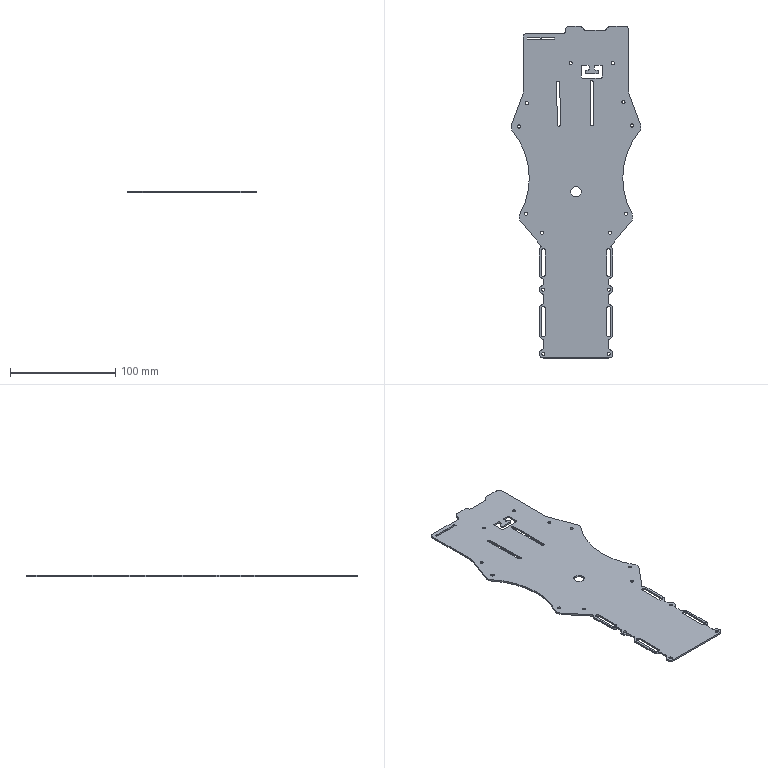Component | SolidWorks | LowerPlate-1 | 1 solid | 168 faces | box 123.18 x 315.5 x 1.6 mm | volume 42538 mm3 | cylinder 111 | plane 57 | commonest cylinder face diameters 3 x33 4 x24 2 x19 8 x18 13 x6 5 x4 140 x3 10 x2
build123d program:
from build123d import *

# Parameters (mm, degrees)
BOSS_EXTRUDE1_DEPTH  = 1.6
FILLET1_R            = 10
FILLET2_R            = 2
BOSS_EXTRUDE2_DEPTH  = 1.6
SKETCH4_R            = 5
SKETCH4_R_2          = 1.5
CUT_EXTRUDE1_2_DEPTH = 1.6
SKETCH5_R            = 1.5
CUT_EXTRUDE2_DEPTH   = 1.6
FILLET3_R            = 1
SKETCH1_W            = 1.25
SKETCH1_H            = 1.5
SKETCH1_W_2          = 1.4
CUT_EXTRUDE1_DEPTH   = 5


with BuildPart() as part:
    # Sketch1_2 → Boss-Extrude1 (new body)
    with BuildSketch(Plane.XY):
        with BuildLine():
            Line((-31, 0), (31, 0))
            ThreePointArc((31, 0), (35, 4), (31, 8))
            Line((31, 8), (31, 18))
            ThreePointArc((31, 18), (33.828, 19.172), (35, 22))
            Line((35, 22), (35, 47))
            ThreePointArc((35, 47), (33.828, 49.828), (31, 51))
            Line((31, 51), (31, 61))
            ThreePointArc((31, 61), (35, 65), (31, 69))
            Line((31, 69), (31, 75.5))
            ThreePointArc((31, 75.5), (33.828, 76.672), (35, 79.5))
            Line((35, 79.5), (35, 101.75))
            ThreePointArc((35, 101.75), (34.694, 103.284), (33.824, 104.583))
            ThreePointArc((33.824, 104.583), (33.237, 105.911), (33.703, 107.286))
            Line((33.703, 107.286), (52.509, 129.698))
            ThreePointArc((52.509, 129.698), (54, 133.254), (53.213, 137.03))
            ThreePointArc((53.213, 137.03), (44.691, 177.172), (60.131, 215.192))
            ThreePointArc((60.131, 215.192), (61.5, 218.215), (61.199, 221.519))
            Line((61.199, 221.519), (50, 252.287))
            Line((50, 252.287), (50, 308))
            Line((50, 308), (-50, 308))
            Line((-50, 308), (-50, 252.287))
            Line((-50, 252.287), (-61.199, 221.519))
            ThreePointArc((-61.199, 221.519), (-61.5, 218.215), (-60.131, 215.192))
            ThreePointArc((-60.131, 215.192), (-44.691, 177.172), (-53.213, 137.03))
            ThreePointArc((-53.213, 137.03), (-54, 133.254), (-52.509, 129.698))
            Line((-52.509, 129.698), (-33.703, 107.286))
            ThreePointArc((-33.703, 107.286), (-33.237, 105.911), (-33.824, 104.583))
            ThreePointArc((-33.824, 104.583), (-34.694, 103.284), (-35, 101.75))
            Line((-35, 101.75), (-35, 79.5))
            ThreePointArc((-35, 79.5), (-33.828, 76.672), (-31, 75.5))
            Line((-31, 75.5), (-31, 69))
            ThreePointArc((-31, 69), (-35, 65), (-31, 61))
            Line((-31, 61), (-31, 51))
            ThreePointArc((-31, 51), (-33.828, 49.828), (-35, 47))
            Line((-35, 47), (-35, 22))
            ThreePointArc((-35, 22), (-33.828, 19.172), (-31, 18))
            Line((-31, 18), (-31, 8))
            ThreePointArc((-31, 8), (-35, 4), (-31, 0))
        make_face()
    extrude(amount=BOSS_EXTRUDE1_DEPTH)

    # Fillet1
    fillet1_edges = [part.edges().sort_by_distance(p)[0] for p in [
        (-50, 252.287, 0.8),
        (50, 252.287, 0.8),
    ]]
    fillet(fillet1_edges, radius=FILLET1_R)

    # Fillet2
    fillet2_edges = [part.edges().sort_by_distance(p)[0] for p in [
        (-31, 8, 0.8),
        (-31, 18, 0.8),
        (-31, 51, 0.8),
        (-31, 61, 0.8),
        (-31, 69, 0.8),
        (-31, 75.5, 0.8),
        (-50, 308, 0.8),
        (50, 308, 0.8),
        (31, 75.5, 0.8),
        (31, 69, 0.8),
        (31, 61, 0.8),
        (31, 51, 0.8),
        (31, 18, 0.8),
        (31, 8, 0.8),
    ]]
    fillet(fillet2_edges, radius=FILLET2_R)

    # Sketch3 → Boss-Extrude2 (add)
    with BuildSketch(Plane.XY.offset(1.6)):
        with BuildLine():
            Line((-6, 315.5), (3, 315.5))
            ThreePointArc((3, 315.5), (5.219, 314.828), (6.692, 313.038))
            ThreePointArc((6.692, 313.038), (7.613, 311.92), (9, 311.5))
            Line((9, 311.5), (27, 311.5))
            ThreePointArc((27, 311.5), (28.387, 311.92), (29.308, 313.038))
            ThreePointArc((29.308, 313.038), (30.781, 314.828), (33, 315.5))
            Line((33, 315.5), (46, 315.5))
            ThreePointArc((46, 315.5), (48.828, 314.328), (50, 311.5))
            Line((50, 311.5), (50, 306))
            ThreePointArc((50, 306), (49.414, 307.414), (48, 308))
            Line((48, 308), (-12.423, 308))
            ThreePointArc((-12.423, 308), (-10.524, 308.874), (-9.952, 310.885))
            ThreePointArc((-9.952, 310.885), (-9.038, 314.102), (-6, 315.5))
        make_face()
    extrude(amount=-BOSS_EXTRUDE2_DEPTH)

    # Sketch4 → Cut-Extrude1_2 (cut)
    with BuildSketch(Plane.XY.offset(1.6)):
        with Locations((0, 158)):
            Circle(SKETCH4_R)
        with Locations((-31, 65)):
            Circle(SKETCH4_R_2)
        with Locations((-31, 4)):
            Circle(SKETCH4_R_2)
        with Locations((-47.464, 137.002)):
            Circle(SKETCH4_R_2)
        with Locations((-32.358, 119)):
            Circle(SKETCH4_R_2)
        with Locations((31, 4)):
            Circle(SKETCH4_R_2)
        with Locations((31, 65)):
            Circle(SKETCH4_R_2)
        with Locations((47.464, 137.002)):
            Circle(SKETCH4_R_2)
        with Locations((32.358, 119)):
            Circle(SKETCH4_R_2)
        with BuildLine():
            Line((-29, 101.75), (-29, 79.5))
            ThreePointArc((-29, 79.5), (-31, 77.5), (-33, 79.5))
            Line((-33, 79.5), (-33, 101.75))
            ThreePointArc((-33, 101.75), (-31, 103.75), (-29, 101.75))
        make_face()
        with BuildLine():
            Line((-29, 47), (-29, 22))
            ThreePointArc((-29, 22), (-31, 20), (-33, 22))
            Line((-33, 22), (-33, 47))
            ThreePointArc((-33, 47), (-31, 49), (-29, 47))
        make_face()
        with BuildLine():
            Line((33, 101.75), (33, 79.5))
            ThreePointArc((33, 79.5), (31, 77.5), (29, 79.5))
            Line((29, 79.5), (29, 101.75))
            ThreePointArc((29, 101.75), (31, 103.75), (33, 101.75))
        make_face()
        with BuildLine():
            Line((33, 47), (33, 22))
            ThreePointArc((33, 22), (31, 20), (29, 22))
            Line((29, 22), (29, 47))
            ThreePointArc((29, 47), (31, 49), (33, 47))
        make_face()
    extrude(amount=-CUT_EXTRUDE1_2_DEPTH, mode=Mode.SUBTRACT)

    # Sketch5 → Cut-Extrude2 (cut)
    with BuildSketch(Plane.XY.offset(1.6)):
        with Locations((45.081, 243.083)):
            Circle(SKETCH5_R)
        with Locations((53.119, 221)):
            Circle(SKETCH5_R)
        with Locations((-5, 280.26)):
            Circle(SKETCH5_R)
        with Locations((35, 280.26)):
            Circle(SKETCH5_R)
        with Locations(Location((-54.309, 219.977, 0), (0, 0, 180))):
            Circle(SKETCH5_R)
        with Locations(Location((-46.694, 242.209, 0), (0, 0, 180))):
            Circle(SKETCH5_R)
        with BuildLine():
            Line((16.51, 262), (16.51, 222))
            ThreePointArc((16.51, 222), (15.01, 220.5), (13.51, 222))
            Line((13.51, 222), (13.51, 262))
            ThreePointArc((13.51, 262), (15.01, 263.5), (16.51, 262))
        make_face()
        with BuildLine():
            Line((-31.339, 302.75), (-22.661, 302.75))
            ThreePointArc((-22.661, 302.75), (-21, 303.5), (-22.661, 304.25))
            Line((-22.661, 304.25), (-31.339, 304.25))
            ThreePointArc((-31.339, 304.25), (-33, 303.5), (-31.339, 302.75))
        make_face()
        Polygon((12.5, 273.5), (12.5, 278), (5, 278), (5, 266), (25, 266), (25, 278), (17.5, 278), (17.5, 273.5), (21, 273.5), (21, 270), (9, 270), (9, 273.5), align=None)
        with BuildLine():
            Line((-44.339, 304.25), (-35.661, 304.25))
            ThreePointArc((-35.661, 304.25), (-34, 303.5), (-35.661, 302.75))
            Line((-35.661, 302.75), (-44.339, 302.75))
            ThreePointArc((-44.339, 302.75), (-46, 303.5), (-44.339, 304.25))
        make_face()
        with BuildLine():
            Line((-18.488, 261.667), (-17.726, 221.674))
            ThreePointArc((-17.726, 221.674), (-16.198, 220.203), (-14.727, 221.731))
            Line((-14.727, 221.731), (-15.489, 261.724))
            ThreePointArc((-15.489, 261.724), (-17.017, 263.195), (-18.488, 261.667))
        make_face()
    extrude(amount=-CUT_EXTRUDE2_DEPTH, mode=Mode.SUBTRACT)

    # Fillet3
    fillet3_edges = [part.edges().sort_by_distance(p)[0] for p in [
        (12.5, 273.5, 0.8),
        (9, 273.5, 0.8),
        (9, 270, 0.8),
        (21, 270, 0.8),
        (21, 273.5, 0.8),
        (17.5, 273.5, 0.8),
        (17.5, 278, 0.8),
        (25, 278, 0.8),
        (25, 266, 0.8),
        (5, 266, 0.8),
        (5, 278, 0.8),
        (12.5, 278, 0.8),
    ]]
    fillet(fillet3_edges, radius=FILLET3_R)

    # Sketch1 → Cut-Extrude1 (cut, symmetric)
    with BuildSketch(Plane.XY):
        with Locations((-45.625, 303.5)):
            Rectangle(SKETCH1_W, SKETCH1_H)
        with Locations((-21.3, 303.5)):
            Rectangle(SKETCH1_W_2, SKETCH1_H)
    extrude(amount=CUT_EXTRUDE1_DEPTH, both=True, mode=Mode.SUBTRACT)


solid = part.part

# Placed as in the assembly
solid = solid.moved(Location((-16.739, -187.575, 1000), (0, 0, 0)))